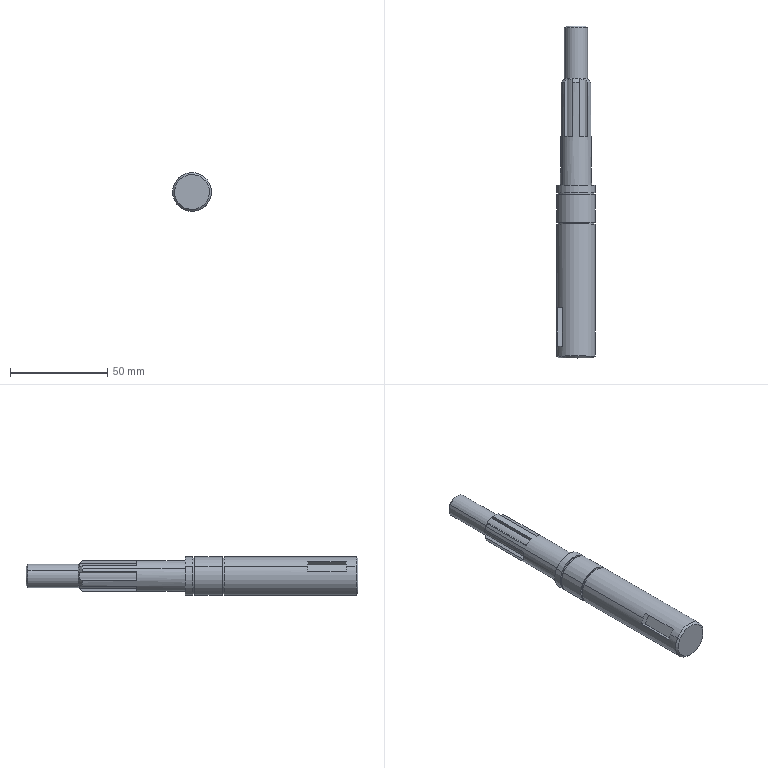Component | SolidWorks | 9-1 | 1 solid | 65 faces | volume 40009 mm3 | plane 33 | cylinder 22 | cone 10 | commonest cylinder face diameters 20 x6 13 x6 18.5 x4 3.15 x2 12 x2 16 x2